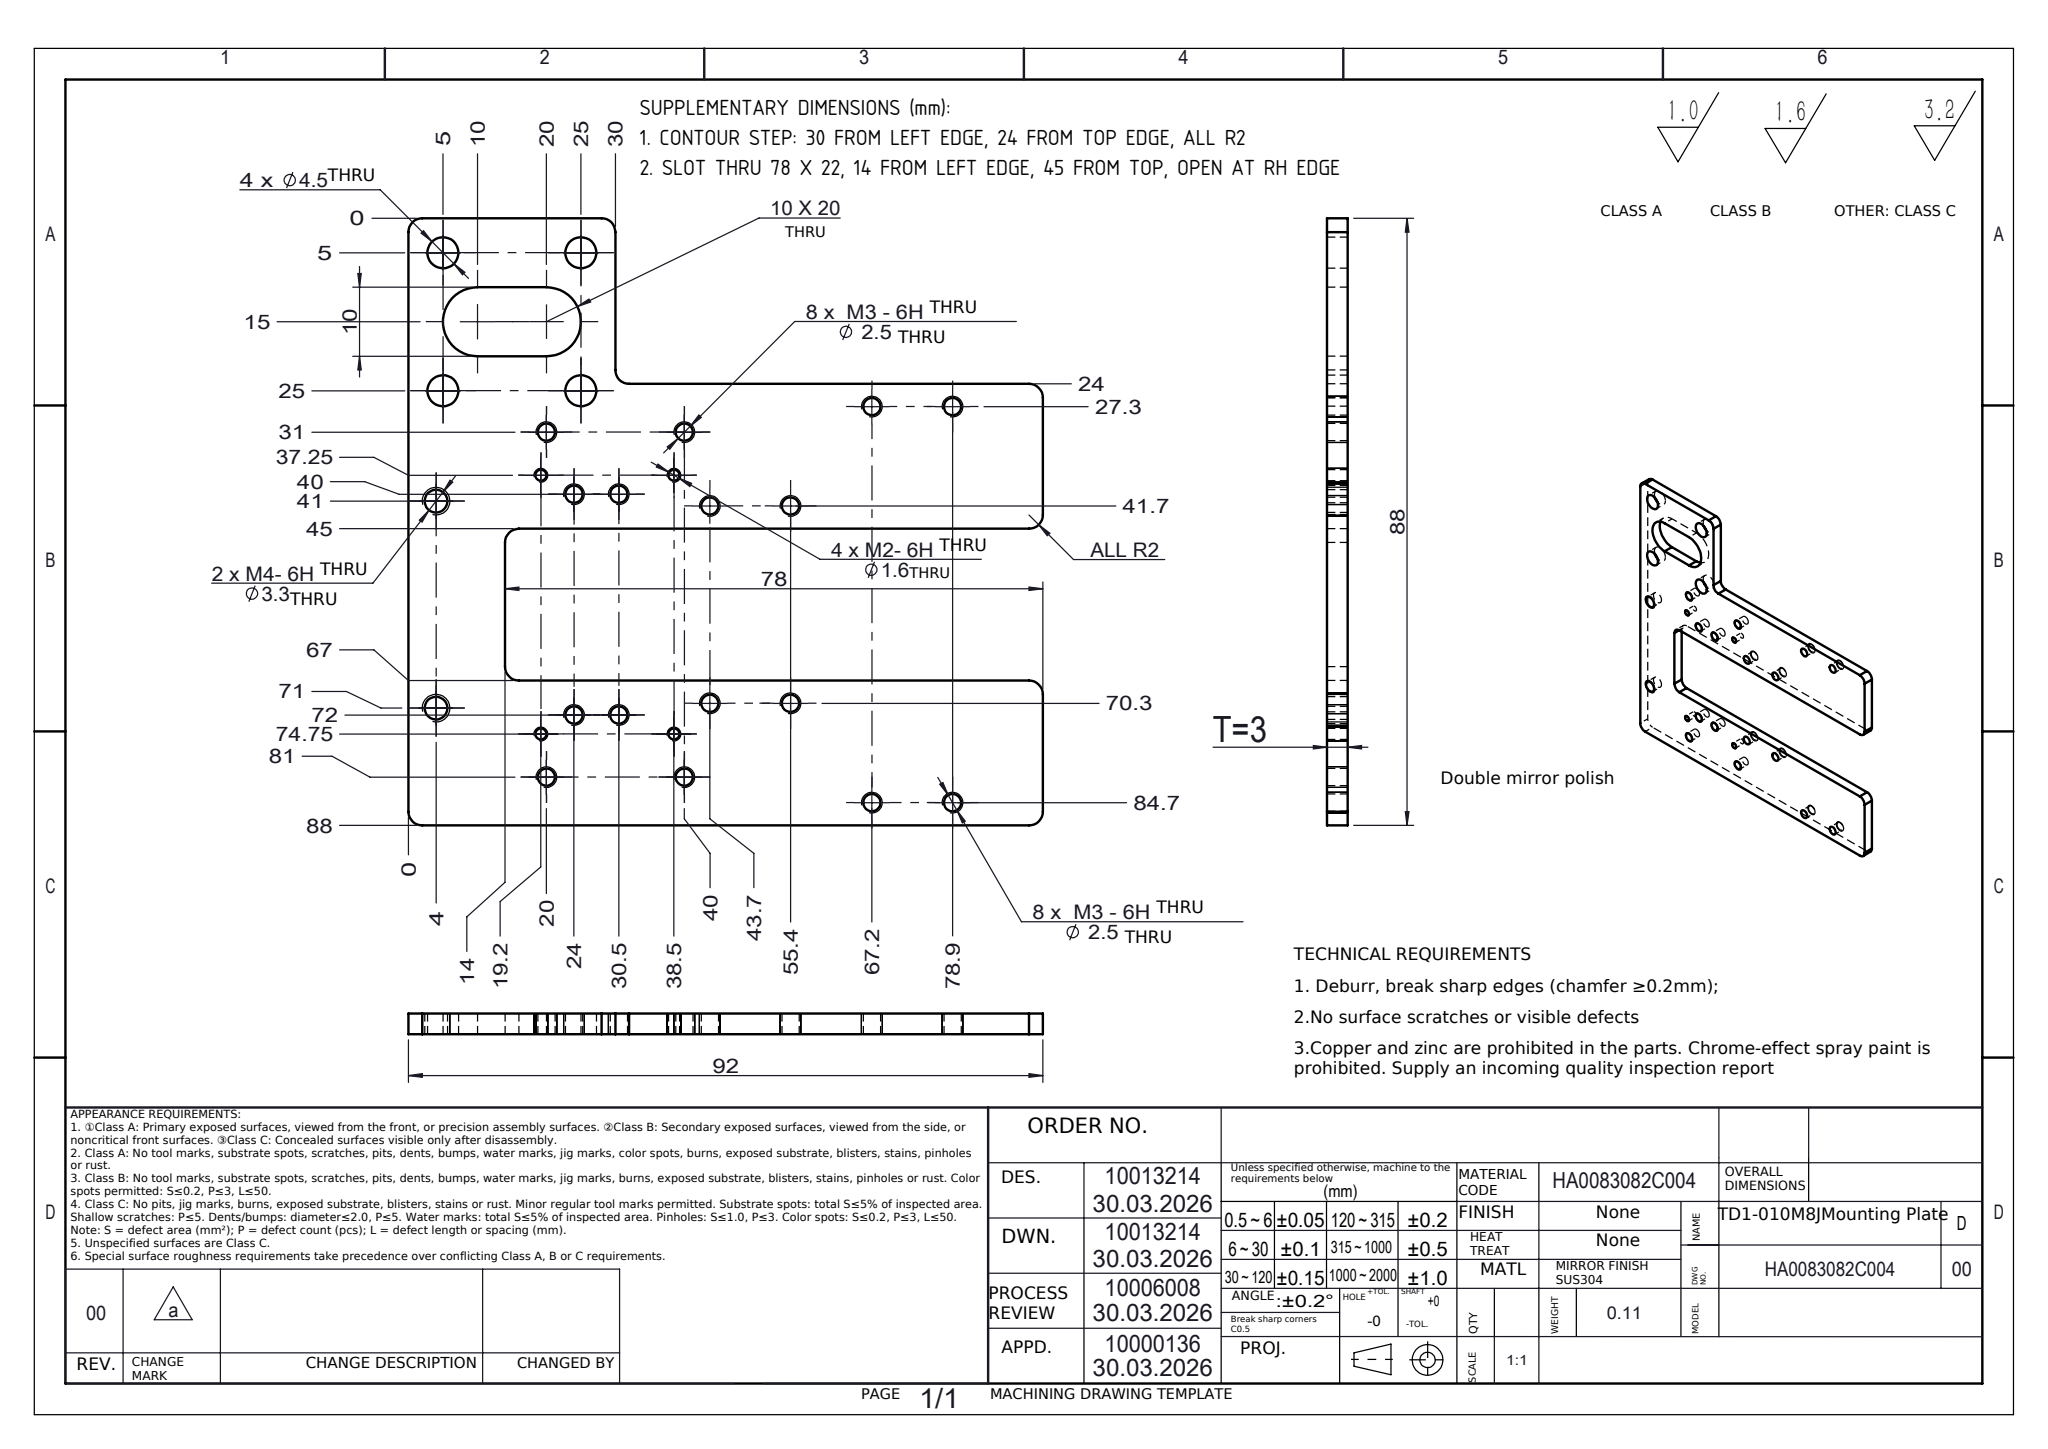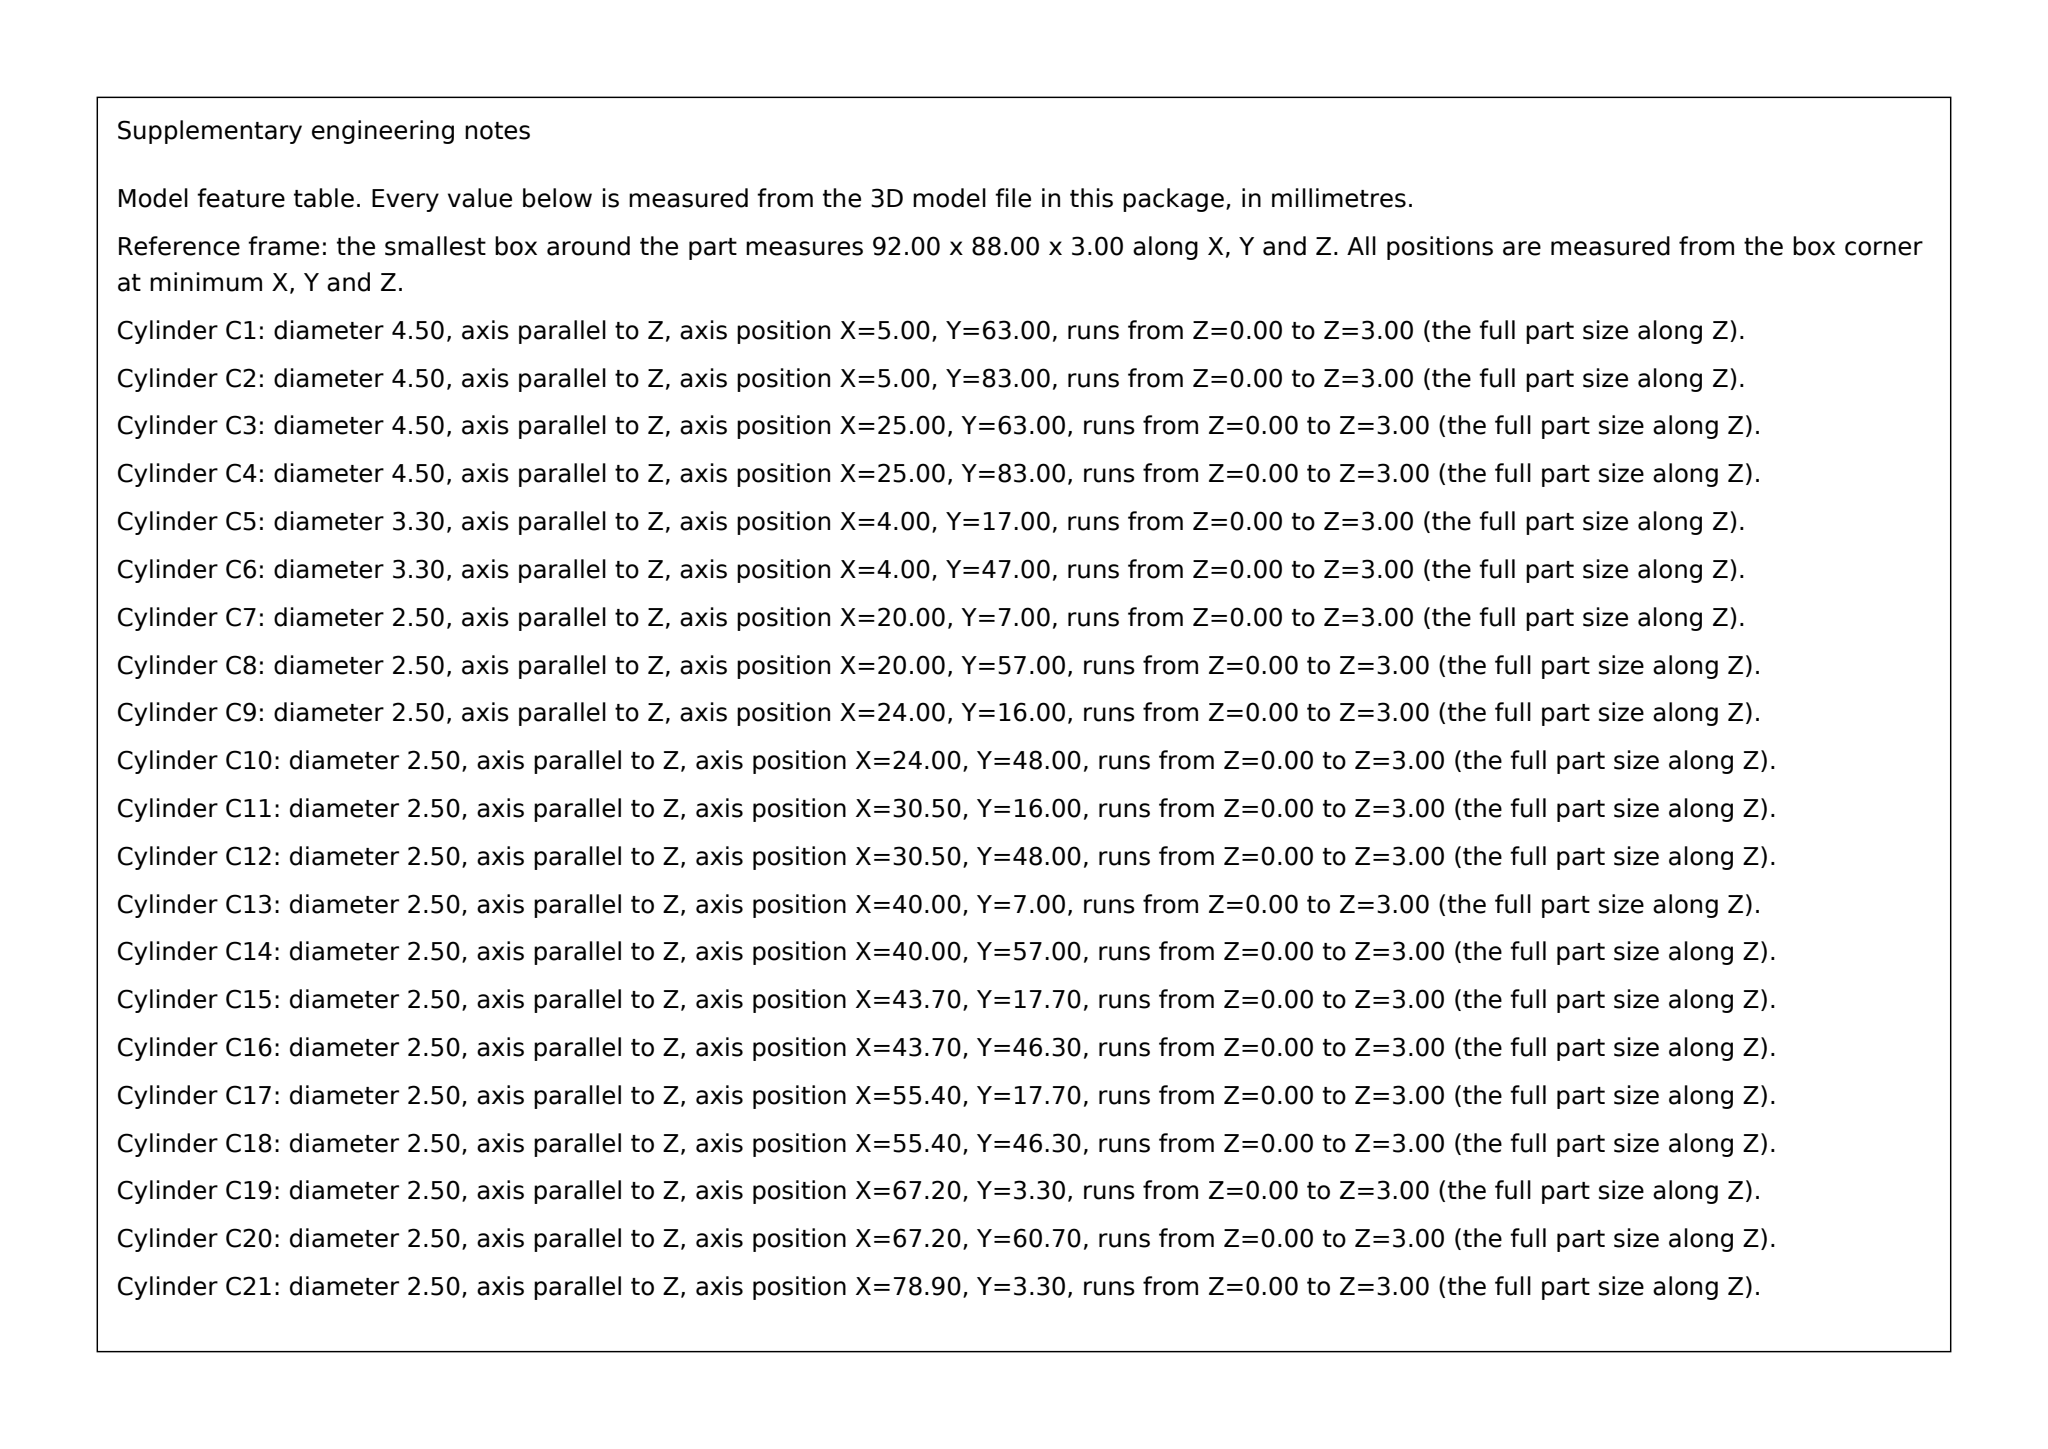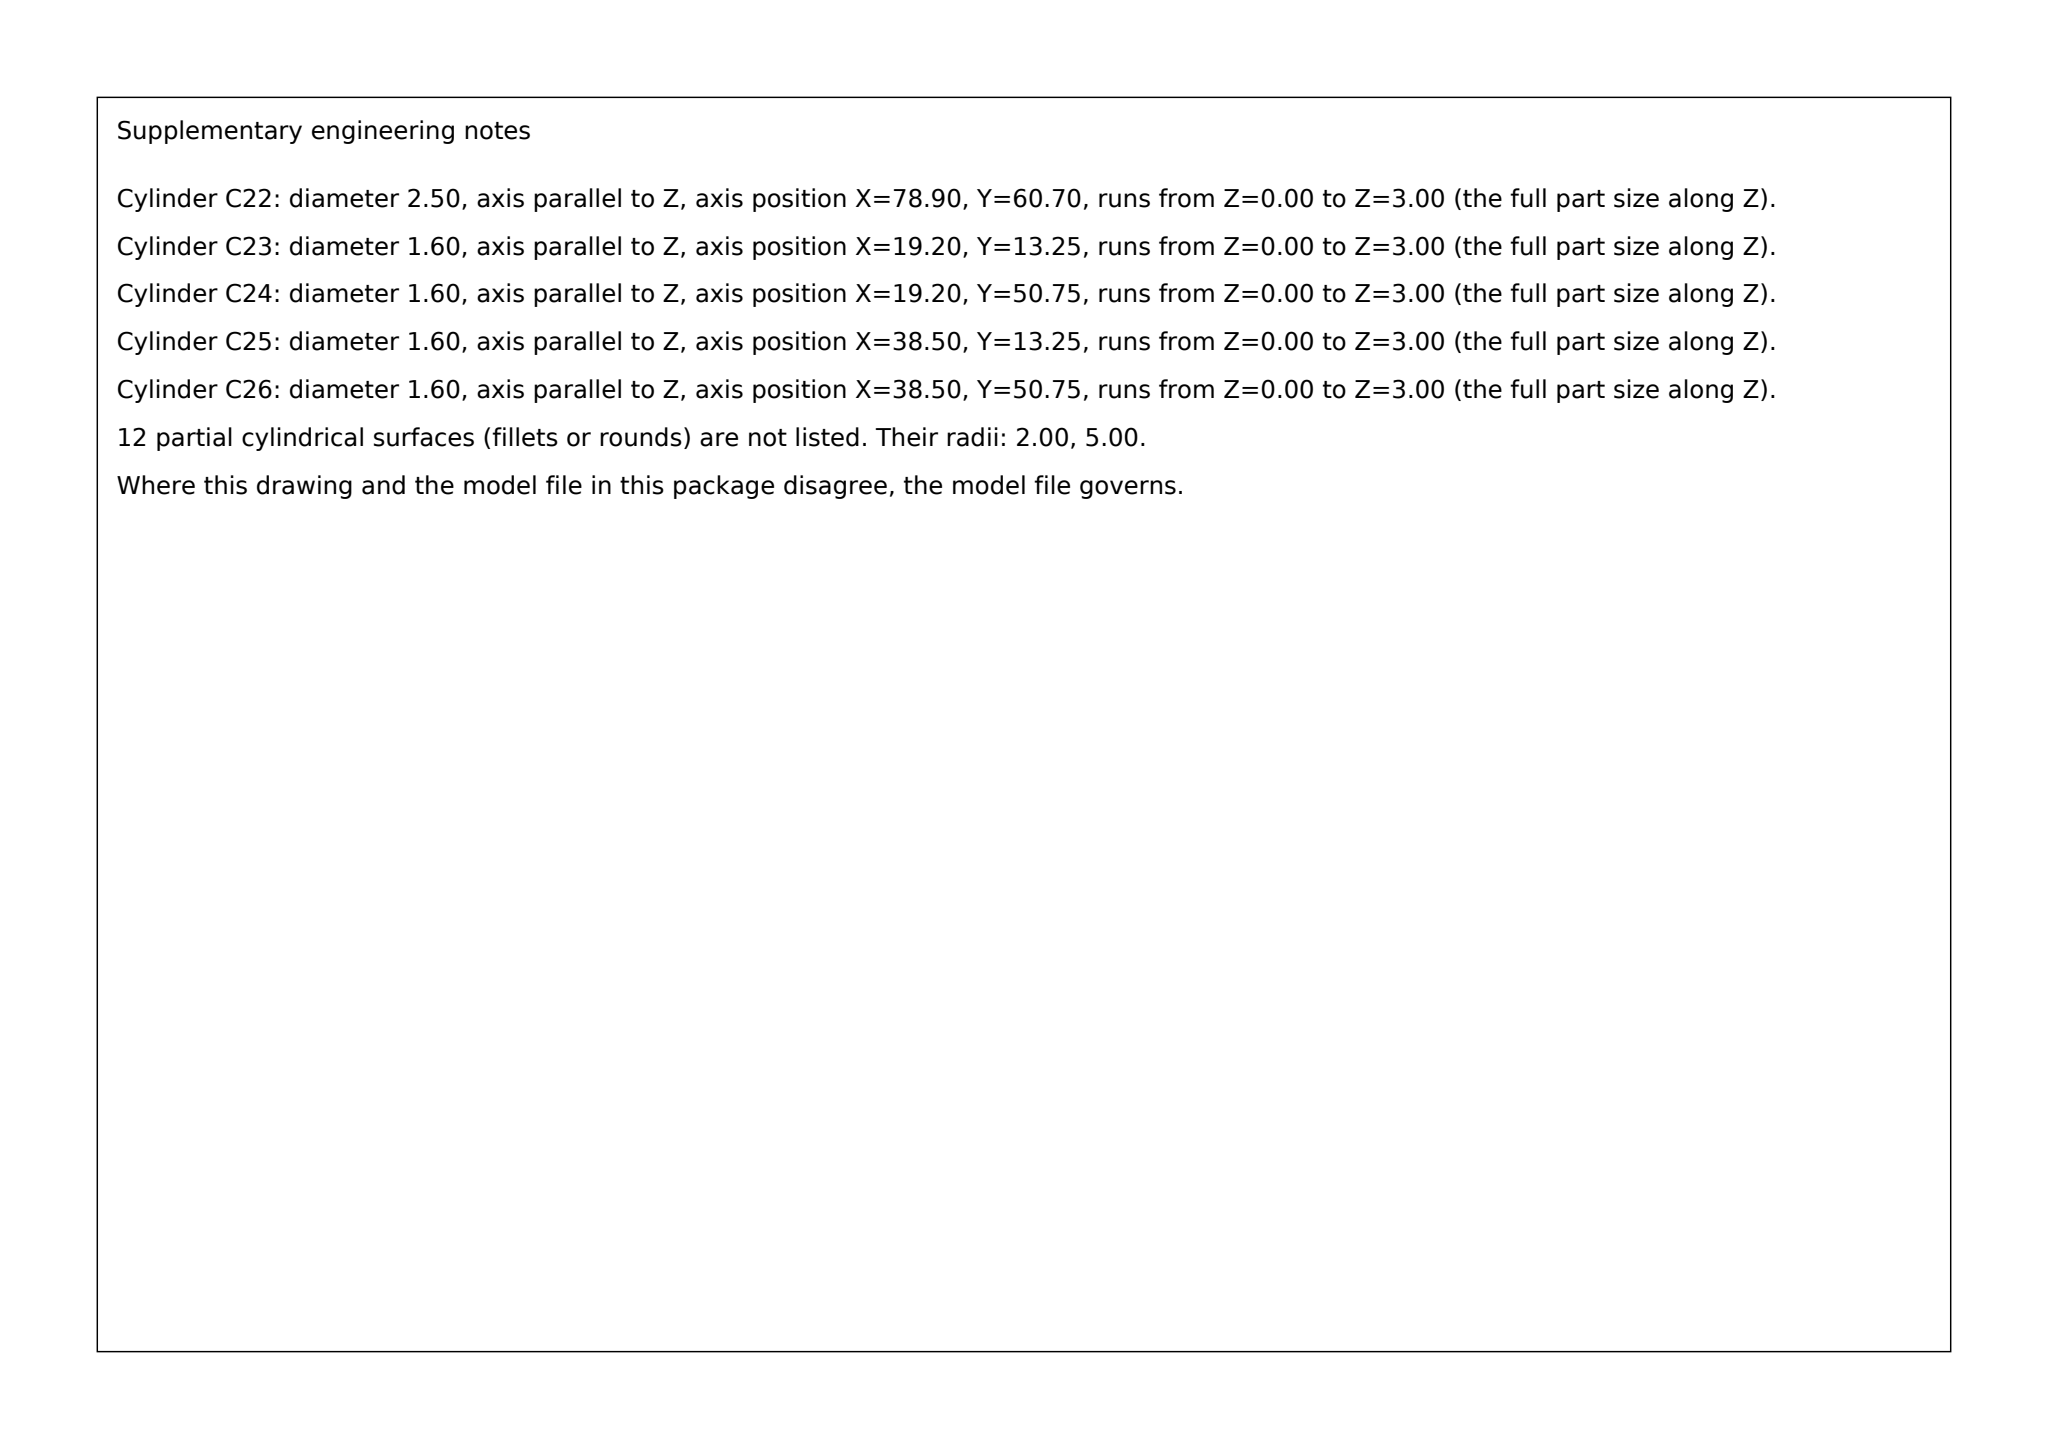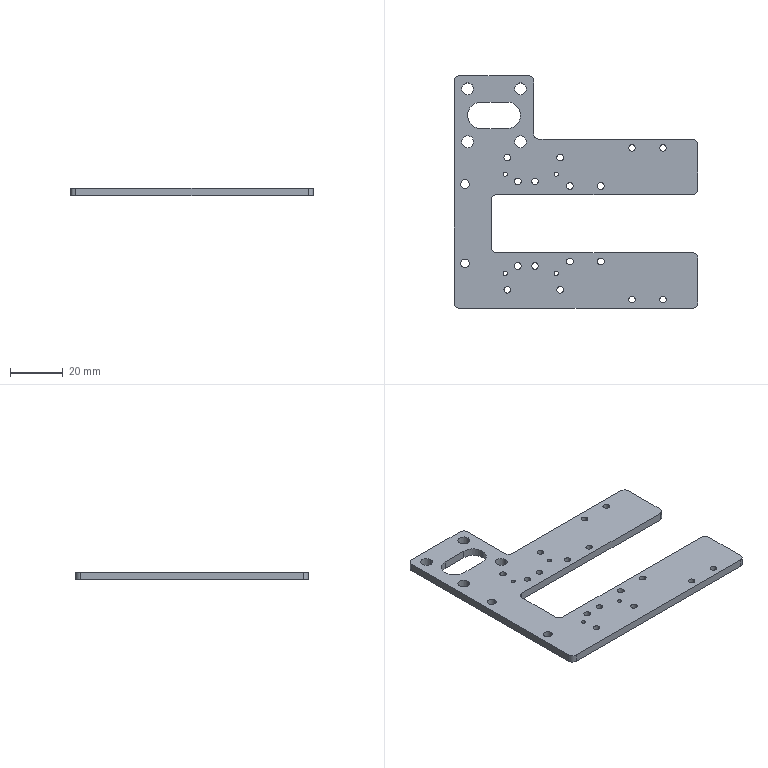Part | SolidWorks | mm | 1 solid | 79 faces | box 92 x 88 x 3 mm | volume 13628 mm3 | cylinder 65 | plane 14 | commonest cylinder face diameters 2.5 x32 4 x10 1.6 x8 4.5 x8 3.3 x4 10 x3
build123d program:
from build123d import *

# Parameters (mm, degrees)
SKETCH1_R           = 1.25
SKETCH1_R_2         = 1.65
SKETCH1_R_3         = 2.25
SKETCH1_R_4         = 0.8
BOSS_EXTRUDE1_DEPTH = 3


with BuildPart() as part:
    # Sketch1 → Boss-Extrude1 (new body)
    with BuildSketch(Plane.XY.offset(3)):
        with BuildLine():
            Line((-44, -44), (44, -44))
            ThreePointArc((44, -44), (45.414, -43.414), (46, -42))
            Line((46, -42), (46, -25))
            ThreePointArc((46, -25), (45.414, -23.586), (44, -23))
            Line((44, -23), (-30, -23))
            ThreePointArc((-30, -23), (-31.414, -22.414), (-32, -21))
            Line((-32, -21), (-32, -3))
            ThreePointArc((-32, -3), (-31.414, -1.586), (-30, -1))
            Line((-30, -1), (44, -1))
            ThreePointArc((44, -1), (45.414, -0.4142), (46, 1))
            Line((46, 1), (46, 18))
            ThreePointArc((46, 18), (45.414, 19.414), (44, 20))
            Line((44, 20), (-14, 20))
            ThreePointArc((-14, 20), (-15.414, 20.586), (-16, 22))
            Line((-16, 22), (-16, 42))
            ThreePointArc((-16, 42), (-16.586, 43.414), (-18, 44))
            Line((-18, 44), (-44, 44))
            ThreePointArc((-44, 44), (-45.414, 43.414), (-46, 42))
            Line((-46, 42), (-46, -42))
            ThreePointArc((-46, -42), (-45.414, -43.414), (-44, -44))
        make_face()
        with Locations(Location((21.2, -40.7, 0), (0, 0, 180))):
            Circle(SKETCH1_R, mode=Mode.SUBTRACT)
        with Locations(Location((-42, 3, 0), (0, 0, 180))):
            Circle(SKETCH1_R_2, mode=Mode.SUBTRACT)
        with Locations(Location((-42, -27, 0), (0, 0, 180))):
            Circle(SKETCH1_R_2, mode=Mode.SUBTRACT)
        with Locations(Location((-41, 19, 0), (0, 0, 180))):
            Circle(SKETCH1_R_3, mode=Mode.SUBTRACT)
        with Locations(Location((-21, 19, 0), (0, 0, 180))):
            Circle(SKETCH1_R_3, mode=Mode.SUBTRACT)
        with Locations(Location((-41, 39, 0), (0, 0, 180))):
            Circle(SKETCH1_R_3, mode=Mode.SUBTRACT)
        with Locations(Location((-21, 39, 0), (0, 0, 180))):
            Circle(SKETCH1_R_3, mode=Mode.SUBTRACT)
        with Locations(Location((-22, 4, 0), (0, 0, 180))):
            Circle(SKETCH1_R, mode=Mode.SUBTRACT)
        with Locations(Location((-15.5, 4, 0), (0, 0, 180))):
            Circle(SKETCH1_R, mode=Mode.SUBTRACT)
        with Locations(Location((-22, -28, 0), (0, 0, 180))):
            Circle(SKETCH1_R, mode=Mode.SUBTRACT)
        with Locations(Location((-15.5, -28, 0), (0, 0, 180))):
            Circle(SKETCH1_R, mode=Mode.SUBTRACT)
        with Locations(Location((-6, -37, 0), (0, 0, 180))):
            Circle(SKETCH1_R, mode=Mode.SUBTRACT)
        with Locations(Location((-26, -37, 0), (0, 0, 180))):
            Circle(SKETCH1_R, mode=Mode.SUBTRACT)
        with Locations(Location((-26, 13, 0), (0, 0, 180))):
            Circle(SKETCH1_R, mode=Mode.SUBTRACT)
        with Locations(Location((-6, 13, 0), (0, 0, 180))):
            Circle(SKETCH1_R, mode=Mode.SUBTRACT)
        with Locations(Location((-26.8, 6.75, 0), (0, 0, 180))):
            Circle(SKETCH1_R_4, mode=Mode.SUBTRACT)
        with Locations(Location((-7.5, 6.75, 0), (0, 0, 180))):
            Circle(SKETCH1_R_4, mode=Mode.SUBTRACT)
        with Locations(Location((-26.8, -30.75, 0), (0, 0, 180))):
            Circle(SKETCH1_R_4, mode=Mode.SUBTRACT)
        with Locations(Location((-7.5, -30.75, 0), (0, 0, 180))):
            Circle(SKETCH1_R_4, mode=Mode.SUBTRACT)
        with Locations(Location((-2.3, -26.3, 0), (0, 0, 180))):
            Circle(SKETCH1_R, mode=Mode.SUBTRACT)
        with Locations(Location((21.2, 16.7, 0), (0, 0, 180))):
            Circle(SKETCH1_R, mode=Mode.SUBTRACT)
        with Locations(Location((-2.3, 2.3, 0), (0, 0, 180))):
            Circle(SKETCH1_R, mode=Mode.SUBTRACT)
        with Locations(Location((32.9, -40.7, 0), (0, 0, 180))):
            Circle(SKETCH1_R, mode=Mode.SUBTRACT)
        with Locations(Location((9.4, -26.3, 0), (0, 0, 180))):
            Circle(SKETCH1_R, mode=Mode.SUBTRACT)
        with Locations(Location((32.9, 16.7, 0), (0, 0, 180))):
            Circle(SKETCH1_R, mode=Mode.SUBTRACT)
        with Locations(Location((9.4, 2.3, 0), (0, 0, 180))):
            Circle(SKETCH1_R, mode=Mode.SUBTRACT)
        with BuildLine():
            Line((-36, 34), (-26, 34))
            ThreePointArc((-26, 34), (-21, 29), (-26, 24))
            Line((-26, 24), (-36, 24))
            ThreePointArc((-36, 24), (-41, 29), (-36, 34))
        make_face(mode=Mode.SUBTRACT)
    extrude(amount=-BOSS_EXTRUDE1_DEPTH)


solid = part.part